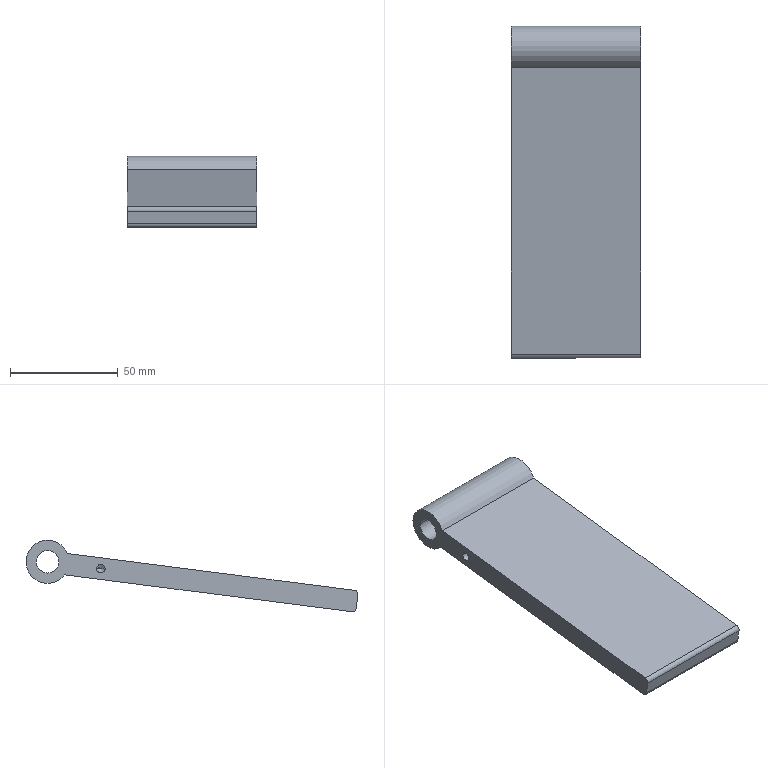Component | SolidWorks | LiftingPlateAssembly-1_LiftingPlate-1 | 1 solid | 18 faces | box 60 x 154.22 x 33.19 mm | volume 94548 mm3 | cylinder 9 | plane 5 | cone 4 | commonest cylinder face diameters 4 x6 10.5 x2 20 x1 | material Plain Carbon Steel
build123d program:
from build123d import *

# Parameters (mm, degrees)
SKETCH1_R             = 5.25
BOSS_EXTRUDE1_DEPTH   = 60
FILLET1_R             = 2
M4_TAPPED_HOLE3_D     = 4
M4_TAPPED_HOLE3_DEPTH = 10.1
M4_TAPPED_HOLE3_TIP   = 1.202
M4_TAPPED_HOLE4_D     = 4
M4_TAPPED_HOLE4_DEPTH = 10.1
M4_TAPPED_HOLE4_TIP   = 1.202


with BuildPart() as part:
    # Sketch1 → Boss-Extrude1 (new body)
    with BuildSketch(Plane.XY):
        with BuildLine():
            Line((-8.66, 5), (-145, 5))
            Line((-145, 5), (-145, -5))
            Line((-145, -5), (-8.66, -5))
            ThreePointArc((-8.66, -5), (10, 0), (-8.66, 5))
        make_face()
        Circle(SKETCH1_R, mode=Mode.SUBTRACT)
    extrude(amount=BOSS_EXTRUDE1_DEPTH)

    # Fillet1
    fillet1_edges = [part.edges().sort_by_distance(p)[0] for p in [
        (-145, 5, 30),
        (-145, -5, 30),
    ]]
    fillet(fillet1_edges, radius=FILLET1_R)

    # M4 Tapped Hole3
    with Locations(Plane.XY.offset(60)):
        with Locations((-25, 0)):
            Hole(M4_TAPPED_HOLE3_D / 2, depth=M4_TAPPED_HOLE3_DEPTH)
            with Locations((0, 0, -(M4_TAPPED_HOLE3_DEPTH + M4_TAPPED_HOLE3_TIP / 2))):  # 118° drill point
                Cone(0, M4_TAPPED_HOLE3_D / 2, M4_TAPPED_HOLE3_TIP, mode=Mode.SUBTRACT)

    # M4 Tapped Hole4
    with Locations(Plane(origin=(0, 0, 0), x_dir=(-1, 0, 0), z_dir=(0, 0, -1))):
        with Locations((25, 0)):
            Hole(M4_TAPPED_HOLE4_D / 2, depth=M4_TAPPED_HOLE4_DEPTH)
            with Locations((0, 0, -(M4_TAPPED_HOLE4_DEPTH + M4_TAPPED_HOLE4_TIP / 2))):  # 118° drill point
                Cone(0, M4_TAPPED_HOLE4_D / 2, M4_TAPPED_HOLE4_TIP, mode=Mode.SUBTRACT)


solid = part.part

# Placed as in the assembly
solid = solid.moved(Location((-220, 2, -65), (-82.682, -90, 0)))
STEP:
#1=CARTESIAN_POINT('',(-9.059,-0.8194,-2.674));
#2=VERTEX_POINT('',#1);
#3=CARTESIAN_POINT('',(-9.059,-0.9756,-2.694));
#4=VERTEX_POINT('',#3);
#5=CARTESIAN_POINT('',(-9.059,-0.8975,-2.684));
#6=DIRECTION('',(1.,0.,-0.));
#7=DIRECTION('',(0.,-0.9919,-0.1274));
#8=AXIS2_PLACEMENT_3D('',#5,#6,#7);
#9=CIRCLE('',#8,0.07874);
#10=EDGE_CURVE('',#2,#4,#9,.T.);
#11=ORIENTED_EDGE('',*,*,#10,.F.);
#12=CARTESIAN_POINT('',(-8.661,-0.8194,-2.674));
#13=VERTEX_POINT('',#12);
#14=CARTESIAN_POINT('',(-8.661,-0.8194,-2.674));
#15=DIRECTION('',(1.,0.,-0.));
#16=VECTOR('',#15,39.37);
#17=LINE('',#14,#16);
#18=EDGE_CURVE('',#2,#13,#17,.T.);
#19=ORIENTED_EDGE('',*,*,#18,.T.);
#20=CARTESIAN_POINT('',(-8.661,-0.9756,-2.694));
#21=VERTEX_POINT('',#20);
#22=CARTESIAN_POINT('',(-8.661,-0.8975,-2.684));
#23=DIRECTION('',(1.,0.,-0.));
#24=DIRECTION('',(0.,-0.9919,-0.1274));
#25=AXIS2_PLACEMENT_3D('',#22,#23,#24);
#26=CIRCLE('',#25,0.07874);
#27=EDGE_CURVE('',#13,#21,#26,.T.);
#28=ORIENTED_EDGE('',*,*,#27,.T.);
#29=CARTESIAN_POINT('',(-8.661,-0.9756,-2.694));
#30=DIRECTION('',(1.,0.,-0.));
#31=VECTOR('',#30,39.37);
#32=LINE('',#29,#31);
#33=EDGE_CURVE('',#4,#21,#32,.T.);
#34=ORIENTED_EDGE('',*,*,#33,.F.);
#35=EDGE_LOOP('',(#11,#19,#28,#34));
#36=FACE_OUTER_BOUND('',#35,.T.);
#37=CARTESIAN_POINT('',(-8.661,-0.8975,-2.684));
#38=DIRECTION('',(1.,0.,-0.));
#39=DIRECTION('',(0.,-0.9919,-0.1274));
#40=AXIS2_PLACEMENT_3D('',#37,#38,#39);
#41=CYLINDRICAL_SURFACE('',#40,0.07874);
#42=ADVANCED_FACE('',(#36),#41,.F.);
#43=CARTESIAN_POINT('',(-9.106,-0.8975,-2.684));
#44=VERTEX_POINT('',#43);
#45=CARTESIAN_POINT('',(-9.059,-0.9756,-2.694));
#46=DIRECTION('',(0.515,-0.8502,-0.1092));
#47=VECTOR('',#46,39.37);
#48=LINE('',#45,#47);
#49=EDGE_CURVE('',#44,#4,#48,.T.);
#50=ORIENTED_EDGE('',*,*,#49,.F.);
#51=CARTESIAN_POINT('',(-9.059,-0.8194,-2.674));
#52=DIRECTION('',(0.515,0.8502,0.1092));
#53=VECTOR('',#52,39.37);
#54=LINE('',#51,#53);
#55=EDGE_CURVE('',#44,#2,#54,.T.);
#56=ORIENTED_EDGE('',*,*,#55,.T.);
#57=ORIENTED_EDGE('',*,*,#10,.T.);
#58=EDGE_LOOP('',(#50,#56,#57));
#59=FACE_OUTER_BOUND('',#58,.T.);
#60=CARTESIAN_POINT('',(-9.059,-0.8975,-2.684));
#61=DIRECTION('',(1.,0.,-0.));
#62=DIRECTION('',(0.,-0.9919,-0.1274));
#63=AXIS2_PLACEMENT_3D('',#60,#61,#62);
#64=CONICAL_SURFACE('',#63,0.07874,1.03);
#65=ADVANCED_FACE('',(#59),#64,.F.);
#66=CARTESIAN_POINT('',(-10.626,-0.9756,-2.694));
#67=VERTEX_POINT('',#66);
#68=CARTESIAN_POINT('',(-10.626,-0.8194,-2.674));
#69=VERTEX_POINT('',#68);
#70=CARTESIAN_POINT('',(-10.626,-0.8975,-2.684));
#71=DIRECTION('',(-1.,-0.,0.));
#72=DIRECTION('',(0.,0.9919,0.1274));
#73=AXIS2_PLACEMENT_3D('',#70,#71,#72);
#74=CIRCLE('',#73,0.07874);
#75=EDGE_CURVE('',#67,#69,#74,.T.);
#76=ORIENTED_EDGE('',*,*,#75,.F.);
#77=CARTESIAN_POINT('',(-11.024,-0.9756,-2.694));
#78=VERTEX_POINT('',#77);
#79=CARTESIAN_POINT('',(-11.024,-0.9756,-2.694));
#80=DIRECTION('',(-1.,-0.,0.));
#81=VECTOR('',#80,39.37);
#82=LINE('',#79,#81);
#83=EDGE_CURVE('',#67,#78,#82,.T.);
#84=ORIENTED_EDGE('',*,*,#83,.T.);
#85=CARTESIAN_POINT('',(-11.024,-0.8194,-2.674));
#86=VERTEX_POINT('',#85);
#87=CARTESIAN_POINT('',(-11.024,-0.8975,-2.684));
#88=DIRECTION('',(-1.,-0.,0.));
#89=DIRECTION('',(0.,0.9919,0.1274));
#90=AXIS2_PLACEMENT_3D('',#87,#88,#89);
#91=CIRCLE('',#90,0.07874);
#92=EDGE_CURVE('',#78,#86,#91,.T.);
#93=ORIENTED_EDGE('',*,*,#92,.T.);
#94=CARTESIAN_POINT('',(-11.024,-0.8194,-2.674));
#95=DIRECTION('',(-1.,-0.,0.));
#96=VECTOR('',#95,39.37);
#97=LINE('',#94,#96);
#98=EDGE_CURVE('',#69,#86,#97,.T.);
#99=ORIENTED_EDGE('',*,*,#98,.F.);
#100=EDGE_LOOP('',(#76,#84,#93,#99));
#101=FACE_OUTER_BOUND('',#100,.T.);
#102=CARTESIAN_POINT('',(-11.024,-0.8975,-2.684));
#103=DIRECTION('',(-1.,-0.,0.));
#104=DIRECTION('',(0.,0.9919,0.1274));
#105=AXIS2_PLACEMENT_3D('',#102,#103,#104);
#106=CYLINDRICAL_SURFACE('',#105,0.07874);
#107=ADVANCED_FACE('',(#101),#106,.F.);
#108=CARTESIAN_POINT('',(-10.579,-0.8975,-2.684));
#109=VERTEX_POINT('',#108);
#110=CARTESIAN_POINT('',(-10.626,-0.8194,-2.674));
#111=DIRECTION('',(-0.515,0.8502,0.1092));
#112=VECTOR('',#111,39.37);
#113=LINE('',#110,#112);
#114=EDGE_CURVE('',#109,#69,#113,.T.);
#115=ORIENTED_EDGE('',*,*,#114,.F.);
#116=CARTESIAN_POINT('',(-10.626,-0.9756,-2.694));
#117=DIRECTION('',(-0.515,-0.8502,-0.1092));
#118=VECTOR('',#117,39.37);
#119=LINE('',#116,#118);
#120=EDGE_CURVE('',#109,#67,#119,.T.);
#121=ORIENTED_EDGE('',*,*,#120,.T.);
#122=ORIENTED_EDGE('',*,*,#75,.T.);
#123=EDGE_LOOP('',(#115,#121,#122));
#124=FACE_OUTER_BOUND('',#123,.T.);
#125=CARTESIAN_POINT('',(-10.626,-0.8975,-2.684));
#126=DIRECTION('',(-1.,-0.,0.));
#127=DIRECTION('',(0.,0.9919,0.1274));
#128=AXIS2_PLACEMENT_3D('',#125,#126,#127);
#129=CONICAL_SURFACE('',#128,0.07874,1.03);
#130=ADVANCED_FACE('',(#124),#129,.F.);
#131=CARTESIAN_POINT('',(-11.024,-0.1263,-2.585));
#132=VERTEX_POINT('',#131);
#133=CARTESIAN_POINT('',(-11.024,0.2837,-2.533));
#134=VERTEX_POINT('',#133);
#135=CARTESIAN_POINT('',(-11.024,0.07874,-2.559));
#136=DIRECTION('',(-1.,-0.,0.));
#137=DIRECTION('',(0.,0.9919,0.1274));
#138=AXIS2_PLACEMENT_3D('',#135,#136,#137);
#139=CIRCLE('',#138,0.2067);
#140=EDGE_CURVE('',#132,#134,#139,.T.);
#141=ORIENTED_EDGE('',*,*,#140,.T.);
#142=CARTESIAN_POINT('',(-8.661,0.2837,-2.533));
#143=VERTEX_POINT('',#142);
#144=CARTESIAN_POINT('',(-11.024,0.2837,-2.533));
#145=DIRECTION('',(1.,0.,-0.));
#146=VECTOR('',#145,39.37);
#147=LINE('',#144,#146);
#148=EDGE_CURVE('',#134,#143,#147,.T.);
#149=ORIENTED_EDGE('',*,*,#148,.T.);
#150=CARTESIAN_POINT('',(-8.661,-0.1263,-2.585));
#151=VERTEX_POINT('',#150);
#152=CARTESIAN_POINT('',(-8.661,0.07874,-2.559));
#153=DIRECTION('',(-1.,-0.,0.));
#154=DIRECTION('',(0.,0.9919,0.1274));
#155=AXIS2_PLACEMENT_3D('',#152,#153,#154);
#156=CIRCLE('',#155,0.2067);
#157=EDGE_CURVE('',#151,#143,#156,.T.);
#158=ORIENTED_EDGE('',*,*,#157,.F.);
#159=CARTESIAN_POINT('',(-11.024,-0.1263,-2.585));
#160=DIRECTION('',(1.,0.,-0.));
#161=VECTOR('',#160,39.37);
#162=LINE('',#159,#161);
#163=EDGE_CURVE('',#132,#151,#162,.T.);
#164=ORIENTED_EDGE('',*,*,#163,.F.);
#165=EDGE_LOOP('',(#141,#149,#158,#164));
#166=FACE_OUTER_BOUND('',#165,.T.);
#167=CARTESIAN_POINT('',(-11.024,0.07874,-2.559));
#168=DIRECTION('',(1.,0.,-0.));
#169=DIRECTION('',(0.,-0.9919,-0.1274));
#170=AXIS2_PLACEMENT_3D('',#167,#168,#169);
#171=CYLINDRICAL_SURFACE('',#170,0.2067);
#172=ADVANCED_FACE('',(#166),#171,.F.);
#173=CARTESIAN_POINT('',(-11.024,-0.8975,-2.684));
#174=DIRECTION('',(-1.,-0.,0.));
#175=DIRECTION('',(0.,0.9919,0.1274));
#176=AXIS2_PLACEMENT_3D('',#173,#174,#175);
#177=CIRCLE('',#176,0.07874);
#178=EDGE_CURVE('',#86,#78,#177,.T.);
#179=ORIENTED_EDGE('',*,*,#178,.F.);
#180=ORIENTED_EDGE('',*,*,#92,.F.);
#181=EDGE_LOOP('',(#179,#180));
#182=FACE_BOUND('',#181,.T.);
#183=CARTESIAN_POINT('',(-11.024,-0.2344,-2.798));
#184=VERTEX_POINT('',#183);
#185=CARTESIAN_POINT('',(-11.024,-5.48,-3.471));
#186=VERTEX_POINT('',#185);
#187=CARTESIAN_POINT('',(-11.024,-0.2344,-2.798));
#188=DIRECTION('',(0.,-0.9919,-0.1274));
#189=VECTOR('',#188,39.37);
#190=LINE('',#187,#189);
#191=EDGE_CURVE('',#184,#186,#190,.T.);
#192=ORIENTED_EDGE('',*,*,#191,.T.);
#193=CARTESIAN_POINT('',(-11.024,-5.568,-3.403));
#194=VERTEX_POINT('',#193);
#195=CARTESIAN_POINT('',(-11.024,-5.49,-3.393));
#196=DIRECTION('',(-1.,-0.,0.));
#197=DIRECTION('',(0.,0.9919,0.1274));
#198=AXIS2_PLACEMENT_3D('',#195,#196,#197);
#199=CIRCLE('',#198,0.07874);
#200=EDGE_CURVE('',#186,#194,#199,.T.);
#201=ORIENTED_EDGE('',*,*,#200,.T.);
#202=CARTESIAN_POINT('',(-11.024,-5.598,-3.169));
#203=VERTEX_POINT('',#202);
#204=CARTESIAN_POINT('',(-11.024,-5.608,-3.091));
#205=DIRECTION('',(0.,-0.1274,0.9919));
#206=VECTOR('',#205,39.37);
#207=LINE('',#204,#206);
#208=EDGE_CURVE('',#194,#203,#207,.T.);
#209=ORIENTED_EDGE('',*,*,#208,.T.);
#210=CARTESIAN_POINT('',(-11.024,-5.53,-3.081));
#211=VERTEX_POINT('',#210);
#212=CARTESIAN_POINT('',(-11.024,-5.52,-3.159));
#213=DIRECTION('',(-1.,-0.,0.));
#214=DIRECTION('',(0.,0.9919,0.1274));
#215=AXIS2_PLACEMENT_3D('',#212,#213,#214);
#216=CIRCLE('',#215,0.07874);
#217=EDGE_CURVE('',#203,#211,#216,.T.);
#218=ORIENTED_EDGE('',*,*,#217,.T.);
#219=CARTESIAN_POINT('',(-11.024,-0.2845,-2.407));
#220=VERTEX_POINT('',#219);
#221=CARTESIAN_POINT('',(-11.024,-0.2845,-2.407));
#222=DIRECTION('',(-0.,0.9919,0.1274));
#223=VECTOR('',#222,39.37);
#224=LINE('',#221,#223);
#225=EDGE_CURVE('',#211,#220,#224,.T.);
#226=ORIENTED_EDGE('',*,*,#225,.T.);
#227=CARTESIAN_POINT('',(-11.024,0.07874,-2.559));
#228=DIRECTION('',(-1.,-0.,0.));
#229=DIRECTION('',(0.,0.9919,0.1274));
#230=AXIS2_PLACEMENT_3D('',#227,#228,#229);
#231=CIRCLE('',#230,0.3937);
#232=EDGE_CURVE('',#220,#184,#231,.T.);
#233=ORIENTED_EDGE('',*,*,#232,.T.);
#234=EDGE_LOOP('',(#192,#201,#209,#218,#226,#233));
#235=FACE_OUTER_BOUND('',#234,.T.);
#236=ORIENTED_EDGE('',*,*,#140,.F.);
#237=CARTESIAN_POINT('',(-11.024,0.07874,-2.559));
#238=DIRECTION('',(-1.,-0.,0.));
#239=DIRECTION('',(0.,0.9919,0.1274));
#240=AXIS2_PLACEMENT_3D('',#237,#238,#239);
#241=CIRCLE('',#240,0.2067);
#242=EDGE_CURVE('',#134,#132,#241,.T.);
#243=ORIENTED_EDGE('',*,*,#242,.F.);
#244=EDGE_LOOP('',(#236,#243));
#245=FACE_BOUND('',#244,.T.);
#246=CARTESIAN_POINT('',(-11.024,0.07874,-2.559));
#247=DIRECTION('',(-1.,-0.,0.));
#248=DIRECTION('',(-0.,0.9919,0.1274));
#249=AXIS2_PLACEMENT_3D('',#246,#247,#248);
#250=PLANE('',#249);
#251=ADVANCED_FACE('',(#182,#235,#245),#250,.T.);
#252=CARTESIAN_POINT('',(-8.661,-0.8975,-2.684));
#253=DIRECTION('',(1.,0.,-0.));
#254=DIRECTION('',(0.,-0.9919,-0.1274));
#255=AXIS2_PLACEMENT_3D('',#252,#253,#254);
#256=CIRCLE('',#255,0.07874);
#257=EDGE_CURVE('',#21,#13,#256,.T.);
#258=ORIENTED_EDGE('',*,*,#257,.F.);
#259=ORIENTED_EDGE('',*,*,#27,.F.);
#260=EDGE_LOOP('',(#258,#259));
#261=FACE_BOUND('',#260,.T.);
#262=CARTESIAN_POINT('',(-8.661,-5.568,-3.403));
#263=VERTEX_POINT('',#262);
#264=CARTESIAN_POINT('',(-8.661,-5.598,-3.169));
#265=VERTEX_POINT('',#264);
#266=CARTESIAN_POINT('',(-8.661,-5.608,-3.091));
#267=DIRECTION('',(0.,-0.1274,0.9919));
#268=VECTOR('',#267,39.37);
#269=LINE('',#266,#268);
#270=EDGE_CURVE('',#263,#265,#269,.T.);
#271=ORIENTED_EDGE('',*,*,#270,.F.);
#272=CARTESIAN_POINT('',(-8.661,-5.48,-3.471));
#273=VERTEX_POINT('',#272);
#274=CARTESIAN_POINT('',(-8.661,-5.49,-3.393));
#275=DIRECTION('',(1.,0.,-0.));
#276=DIRECTION('',(0.,0.9919,0.1274));
#277=AXIS2_PLACEMENT_3D('',#274,#275,#276);
#278=CIRCLE('',#277,0.07874);
#279=EDGE_CURVE('',#263,#273,#278,.T.);
#280=ORIENTED_EDGE('',*,*,#279,.T.);
#281=CARTESIAN_POINT('',(-8.661,-0.2344,-2.798));
#282=VERTEX_POINT('',#281);
#283=CARTESIAN_POINT('',(-8.661,-0.2344,-2.798));
#284=DIRECTION('',(0.,-0.9919,-0.1274));
#285=VECTOR('',#284,39.37);
#286=LINE('',#283,#285);
#287=EDGE_CURVE('',#282,#273,#286,.T.);
#288=ORIENTED_EDGE('',*,*,#287,.F.);
#289=CARTESIAN_POINT('',(-8.661,-0.2845,-2.407));
#290=VERTEX_POINT('',#289);
#291=CARTESIAN_POINT('',(-8.661,0.07874,-2.559));
#292=DIRECTION('',(-1.,-0.,0.));
#293=DIRECTION('',(0.,0.9919,0.1274));
#294=AXIS2_PLACEMENT_3D('',#291,#292,#293);
#295=CIRCLE('',#294,0.3937);
#296=EDGE_CURVE('',#290,#282,#295,.T.);
#297=ORIENTED_EDGE('',*,*,#296,.F.);
#298=CARTESIAN_POINT('',(-8.661,-5.53,-3.081));
#299=VERTEX_POINT('',#298);
#300=CARTESIAN_POINT('',(-8.661,-0.2845,-2.407));
#301=DIRECTION('',(-0.,0.9919,0.1274));
#302=VECTOR('',#301,39.37);
#303=LINE('',#300,#302);
#304=EDGE_CURVE('',#299,#290,#303,.T.);
#305=ORIENTED_EDGE('',*,*,#304,.F.);
#306=CARTESIAN_POINT('',(-8.661,-5.52,-3.159));
#307=DIRECTION('',(1.,0.,-0.));
#308=DIRECTION('',(0.,0.9919,0.1274));
#309=AXIS2_PLACEMENT_3D('',#306,#307,#308);
#310=CIRCLE('',#309,0.07874);
#311=EDGE_CURVE('',#299,#265,#310,.T.);
#312=ORIENTED_EDGE('',*,*,#311,.T.);
#313=EDGE_LOOP('',(#271,#280,#288,#297,#305,#312));
#314=FACE_OUTER_BOUND('',#313,.T.);
#315=ORIENTED_EDGE('',*,*,#157,.T.);
#316=CARTESIAN_POINT('',(-8.661,0.07874,-2.559));
#317=DIRECTION('',(-1.,-0.,0.));
#318=DIRECTION('',(0.,0.9919,0.1274));
#319=AXIS2_PLACEMENT_3D('',#316,#317,#318);
#320=CIRCLE('',#319,0.2067);
#321=EDGE_CURVE('',#143,#151,#320,.T.);
#322=ORIENTED_EDGE('',*,*,#321,.T.);
#323=EDGE_LOOP('',(#315,#322));
#324=FACE_BOUND('',#323,.T.);
#325=CARTESIAN_POINT('',(-8.661,0.07874,-2.559));
#326=DIRECTION('',(-1.,-0.,0.));
#327=DIRECTION('',(-0.,0.9919,0.1274));
#328=AXIS2_PLACEMENT_3D('',#325,#326,#327);
#329=PLANE('',#328);
#330=ADVANCED_FACE('',(#261,#314,#324),#329,.F.);
#331=ORIENTED_EDGE('',*,*,#208,.F.);
#332=CARTESIAN_POINT('',(-11.024,-5.568,-3.403));
#333=DIRECTION('',(1.,0.,-0.));
#334=VECTOR('',#333,39.37);
#335=LINE('',#332,#334);
#336=EDGE_CURVE('',#194,#263,#335,.T.);
#337=ORIENTED_EDGE('',*,*,#336,.T.);
#338=ORIENTED_EDGE('',*,*,#270,.T.);
#339=CARTESIAN_POINT('',(-11.024,-5.598,-3.169));
#340=DIRECTION('',(-1.,-0.,0.));
#341=VECTOR('',#340,39.37);
#342=LINE('',#339,#341);
#343=EDGE_CURVE('',#265,#203,#342,.T.);
#344=ORIENTED_EDGE('',*,*,#343,.T.);
#345=EDGE_LOOP('',(#331,#337,#338,#344));
#346=FACE_OUTER_BOUND('',#345,.T.);
#347=CARTESIAN_POINT('',(-11.024,-5.608,-3.091));
#348=DIRECTION('',(-0.,0.9919,0.1274));
#349=DIRECTION('',(-0.,0.1274,-0.9919));
#350=AXIS2_PLACEMENT_3D('',#347,#348,#349);
#351=PLANE('',#350);
#352=ADVANCED_FACE('',(#346),#351,.F.);
#353=ORIENTED_EDGE('',*,*,#225,.F.);
#354=CARTESIAN_POINT('',(-11.024,-5.53,-3.081));
#355=DIRECTION('',(1.,0.,-0.));
#356=VECTOR('',#355,39.37);
#357=LINE('',#354,#356);
#358=EDGE_CURVE('',#211,#299,#357,.T.);
#359=ORIENTED_EDGE('',*,*,#358,.T.);
#360=ORIENTED_EDGE('',*,*,#304,.T.);
#361=CARTESIAN_POINT('',(-11.024,-0.2845,-2.407));
#362=DIRECTION('',(1.,0.,-0.));
#363=VECTOR('',#362,39.37);
#364=LINE('',#361,#363);
#365=EDGE_CURVE('',#220,#290,#364,.T.);
#366=ORIENTED_EDGE('',*,*,#365,.F.);
#367=EDGE_LOOP('',(#353,#359,#360,#366));
#368=FACE_OUTER_BOUND('',#367,.T.);
#369=CARTESIAN_POINT('',(-11.024,-0.2845,-2.407));
#370=DIRECTION('',(-0.,0.1274,-0.9919));
#371=DIRECTION('',(0.,-0.9919,-0.1274));
#372=AXIS2_PLACEMENT_3D('',#369,#370,#371);
#373=PLANE('',#372);
#374=ADVANCED_FACE('',(#368),#373,.F.);
#375=ORIENTED_EDGE('',*,*,#296,.T.);
#376=CARTESIAN_POINT('',(-11.024,-0.2344,-2.798));
#377=DIRECTION('',(1.,0.,-0.));
#378=VECTOR('',#377,39.37);
#379=LINE('',#376,#378);
#380=EDGE_CURVE('',#184,#282,#379,.T.);
#381=ORIENTED_EDGE('',*,*,#380,.F.);
#382=ORIENTED_EDGE('',*,*,#232,.F.);
#383=ORIENTED_EDGE('',*,*,#365,.T.);
#384=EDGE_LOOP('',(#375,#381,#382,#383));
#385=FACE_OUTER_BOUND('',#384,.T.);
#386=CARTESIAN_POINT('',(-11.024,0.07874,-2.559));
#387=DIRECTION('',(1.,0.,-0.));
#388=DIRECTION('',(0.,-0.9919,-0.1274));
#389=AXIS2_PLACEMENT_3D('',#386,#387,#388);
#390=CYLINDRICAL_SURFACE('',#389,0.3937);
#391=ADVANCED_FACE('',(#385),#390,.T.);
#392=ORIENTED_EDGE('',*,*,#287,.T.);
#393=CARTESIAN_POINT('',(-11.024,-5.48,-3.471));
#394=DIRECTION('',(-1.,-0.,0.));
#395=VECTOR('',#394,39.37);
#396=LINE('',#393,#395);
#397=EDGE_CURVE('',#273,#186,#396,.T.);
#398=ORIENTED_EDGE('',*,*,#397,.T.);
#399=ORIENTED_EDGE('',*,*,#191,.F.);
#400=ORIENTED_EDGE('',*,*,#380,.T.);
#401=EDGE_LOOP('',(#392,#398,#399,#400));
#402=FACE_OUTER_BOUND('',#401,.T.);
#403=CARTESIAN_POINT('',(-11.024,-0.2344,-2.798));
#404=DIRECTION('',(0.,-0.1274,0.9919));
#405=DIRECTION('',(-0.,0.9919,0.1274));
#406=AXIS2_PLACEMENT_3D('',#403,#404,#405);
#407=PLANE('',#406);
#408=ADVANCED_FACE('',(#402),#407,.F.);
#409=ORIENTED_EDGE('',*,*,#148,.F.);
#410=ORIENTED_EDGE('',*,*,#242,.T.);
#411=ORIENTED_EDGE('',*,*,#163,.T.);
#412=ORIENTED_EDGE('',*,*,#321,.F.);
#413=EDGE_LOOP('',(#409,#410,#411,#412));
#414=FACE_OUTER_BOUND('',#413,.T.);
#415=CARTESIAN_POINT('',(-11.024,0.07874,-2.559));
#416=DIRECTION('',(1.,0.,-0.));
#417=DIRECTION('',(0.,-0.9919,-0.1274));
#418=AXIS2_PLACEMENT_3D('',#415,#416,#417);
#419=CYLINDRICAL_SURFACE('',#418,0.2067);
#420=ADVANCED_FACE('',(#414),#419,.F.);
#421=ORIENTED_EDGE('',*,*,#200,.F.);
#422=ORIENTED_EDGE('',*,*,#397,.F.);
#423=ORIENTED_EDGE('',*,*,#279,.F.);
#424=ORIENTED_EDGE('',*,*,#336,.F.);
#425=EDGE_LOOP('',(#421,#422,#423,#424));
#426=FACE_OUTER_BOUND('',#425,.T.);
#427=CARTESIAN_POINT('',(-11.024,-5.49,-3.393));
#428=DIRECTION('',(1.,0.,-0.));
#429=DIRECTION('',(0.,-0.9919,-0.1274));
#430=AXIS2_PLACEMENT_3D('',#427,#428,#429);
#431=CYLINDRICAL_SURFACE('',#430,0.07874);
#432=ADVANCED_FACE('',(#426),#431,.T.);
#433=ORIENTED_EDGE('',*,*,#217,.F.);
#434=ORIENTED_EDGE('',*,*,#343,.F.);
#435=ORIENTED_EDGE('',*,*,#311,.F.);
#436=ORIENTED_EDGE('',*,*,#358,.F.);
#437=EDGE_LOOP('',(#433,#434,#435,#436));
#438=FACE_OUTER_BOUND('',#437,.T.);
#439=CARTESIAN_POINT('',(-11.024,-5.52,-3.159));
#440=DIRECTION('',(1.,0.,-0.));
#441=DIRECTION('',(0.,-0.9919,-0.1274));
#442=AXIS2_PLACEMENT_3D('',#439,#440,#441);
#443=CYLINDRICAL_SURFACE('',#442,0.07874);
#444=ADVANCED_FACE('',(#438),#443,.T.);
#445=ORIENTED_EDGE('',*,*,#120,.F.);
#446=ORIENTED_EDGE('',*,*,#114,.T.);
#447=CARTESIAN_POINT('',(-10.626,-0.8975,-2.684));
#448=DIRECTION('',(-1.,-0.,0.));
#449=DIRECTION('',(0.,0.9919,0.1274));
#450=AXIS2_PLACEMENT_3D('',#447,#448,#449);
#451=CIRCLE('',#450,0.07874);
#452=EDGE_CURVE('',#69,#67,#451,.T.);
#453=ORIENTED_EDGE('',*,*,#452,.T.);
#454=EDGE_LOOP('',(#445,#446,#453));
#455=FACE_OUTER_BOUND('',#454,.T.);
#456=CARTESIAN_POINT('',(-10.626,-0.8975,-2.684));
#457=DIRECTION('',(-1.,-0.,0.));
#458=DIRECTION('',(0.,0.9919,0.1274));
#459=AXIS2_PLACEMENT_3D('',#456,#457,#458);
#460=CONICAL_SURFACE('',#459,0.07874,1.03);
#461=ADVANCED_FACE('',(#455),#460,.F.);
#462=ORIENTED_EDGE('',*,*,#83,.F.);
#463=ORIENTED_EDGE('',*,*,#452,.F.);
#464=ORIENTED_EDGE('',*,*,#98,.T.);
#465=ORIENTED_EDGE('',*,*,#178,.T.);
#466=EDGE_LOOP('',(#462,#463,#464,#465));
#467=FACE_OUTER_BOUND('',#466,.T.);
#468=CARTESIAN_POINT('',(-11.024,-0.8975,-2.684));
#469=DIRECTION('',(-1.,-0.,0.));
#470=DIRECTION('',(0.,0.9919,0.1274));
#471=AXIS2_PLACEMENT_3D('',#468,#469,#470);
#472=CYLINDRICAL_SURFACE('',#471,0.07874);
#473=ADVANCED_FACE('',(#467),#472,.F.);
#474=ORIENTED_EDGE('',*,*,#55,.F.);
#475=ORIENTED_EDGE('',*,*,#49,.T.);
#476=CARTESIAN_POINT('',(-9.059,-0.8975,-2.684));
#477=DIRECTION('',(1.,0.,-0.));
#478=DIRECTION('',(0.,-0.9919,-0.1274));
#479=AXIS2_PLACEMENT_3D('',#476,#477,#478);
#480=CIRCLE('',#479,0.07874);
#481=EDGE_CURVE('',#4,#2,#480,.T.);
#482=ORIENTED_EDGE('',*,*,#481,.T.);
#483=EDGE_LOOP('',(#474,#475,#482));
#484=FACE_OUTER_BOUND('',#483,.T.);
#485=CARTESIAN_POINT('',(-9.059,-0.8975,-2.684));
#486=DIRECTION('',(1.,0.,-0.));
#487=DIRECTION('',(0.,-0.9919,-0.1274));
#488=AXIS2_PLACEMENT_3D('',#485,#486,#487);
#489=CONICAL_SURFACE('',#488,0.07874,1.03);
#490=ADVANCED_FACE('',(#484),#489,.F.);
#491=ORIENTED_EDGE('',*,*,#18,.F.);
#492=ORIENTED_EDGE('',*,*,#481,.F.);
#493=ORIENTED_EDGE('',*,*,#33,.T.);
#494=ORIENTED_EDGE('',*,*,#257,.T.);
#495=EDGE_LOOP('',(#491,#492,#493,#494));
#496=FACE_OUTER_BOUND('',#495,.T.);
#497=CARTESIAN_POINT('',(-8.661,-0.8975,-2.684));
#498=DIRECTION('',(1.,0.,-0.));
#499=DIRECTION('',(0.,-0.9919,-0.1274));
#500=AXIS2_PLACEMENT_3D('',#497,#498,#499);
#501=CYLINDRICAL_SURFACE('',#500,0.07874);
#502=ADVANCED_FACE('',(#496),#501,.F.);
#503=CLOSED_SHELL('',(#42,#65,#107,#130,#172,#251,#330,#352,#374,#391,#408,#420,#432,#444,#461,#473,#490,#502));
#504=MANIFOLD_SOLID_BREP('',#503);
#505=CARTESIAN_POINT('',(0.,0.,0.));
#506=DIRECTION('',(0.,0.,1.));
#507=DIRECTION('',(1.,0.,0.));
#508=AXIS2_PLACEMENT_3D('',#505,#506,#507);
#509=(LENGTH_UNIT()NAMED_UNIT(*)SI_UNIT($,.METRE.));
#510=LENGTH_MEASURE_WITH_UNIT(LENGTH_MEASURE(0.0254),#509);
#511=DIMENSIONAL_EXPONENTS(1.,0.,0.,0.,0.,0.,0.);
#512=(CONVERSION_BASED_UNIT('',#510)LENGTH_UNIT()NAMED_UNIT(#511));
#513=UNCERTAINTY_MEASURE_WITH_UNIT(LENGTH_MEASURE(0.00001),#512,'','');
#514=(NAMED_UNIT(*)PLANE_ANGLE_UNIT()SI_UNIT($,.RADIAN.));
#515=(NAMED_UNIT(*)SI_UNIT($,.STERADIAN.)SOLID_ANGLE_UNIT());
#516=(GEOMETRIC_REPRESENTATION_CONTEXT(3)GLOBAL_UNCERTAINTY_ASSIGNED_CONTEXT((#513))GLOBAL_UNIT_ASSIGNED_CONTEXT((#512,#514,#515))REPRESENTATION_CONTEXT('',''));
#517=ADVANCED_BREP_SHAPE_REPRESENTATION('',(#504,#508),#516);
#518=COLOUR_RGB('',0.7922,0.8196,0.9333);
#519=FILL_AREA_STYLE_COLOUR('',#518);
#520=FILL_AREA_STYLE('',(#519));
#521=SURFACE_STYLE_FILL_AREA(#520);
#522=SURFACE_SIDE_STYLE('',(#521));
#523=SURFACE_STYLE_USAGE(.BOTH.,#522);
#524=PRESENTATION_STYLE_ASSIGNMENT((#523));
#525=STYLED_ITEM('',(#524),#504);
#526=PRESENTATION_LAYER_ASSIGNMENT('','',(#525));
#527=(LENGTH_UNIT()NAMED_UNIT(*)SI_UNIT($,.METRE.));
#528=LENGTH_MEASURE_WITH_UNIT(LENGTH_MEASURE(0.0254),#527);
#529=DIMENSIONAL_EXPONENTS(1.,0.,0.,0.,0.,0.,0.);
#530=(CONVERSION_BASED_UNIT('',#528)LENGTH_UNIT()NAMED_UNIT(#529));
#531=UNCERTAINTY_MEASURE_WITH_UNIT(LENGTH_MEASURE(0.00001),#530,'','');
#532=(NAMED_UNIT(*)PLANE_ANGLE_UNIT()SI_UNIT($,.RADIAN.));
#533=(NAMED_UNIT(*)SI_UNIT($,.STERADIAN.)SOLID_ANGLE_UNIT());
#534=(GEOMETRIC_REPRESENTATION_CONTEXT(3)GLOBAL_UNCERTAINTY_ASSIGNED_CONTEXT((#531))GLOBAL_UNIT_ASSIGNED_CONTEXT((#530,#532,#533))REPRESENTATION_CONTEXT('',''));
#535=MECHANICAL_DESIGN_GEOMETRIC_PRESENTATION_REPRESENTATION('',(#525),#534);